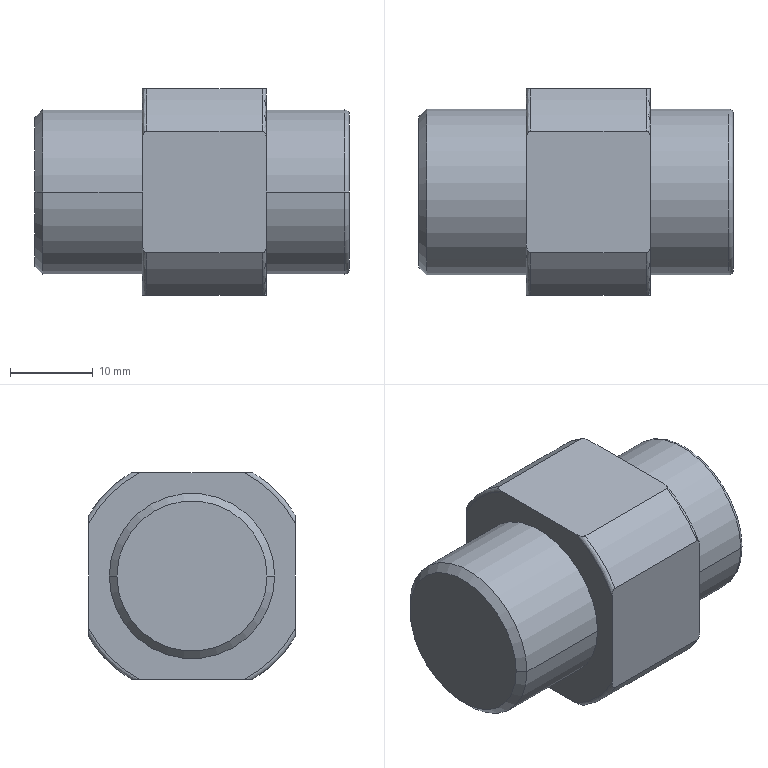Component | SolidWorks | RMS_20X400_03-1_RMS20X50_FCV-1 | 1 solid | 44 faces | volume 12617 mm3 | cylinder 14 | plane 14 | torus 10 | cone 6 | commonest cylinder face diameters 20 x4 29 x4 3 x2 10 x2 11 x2